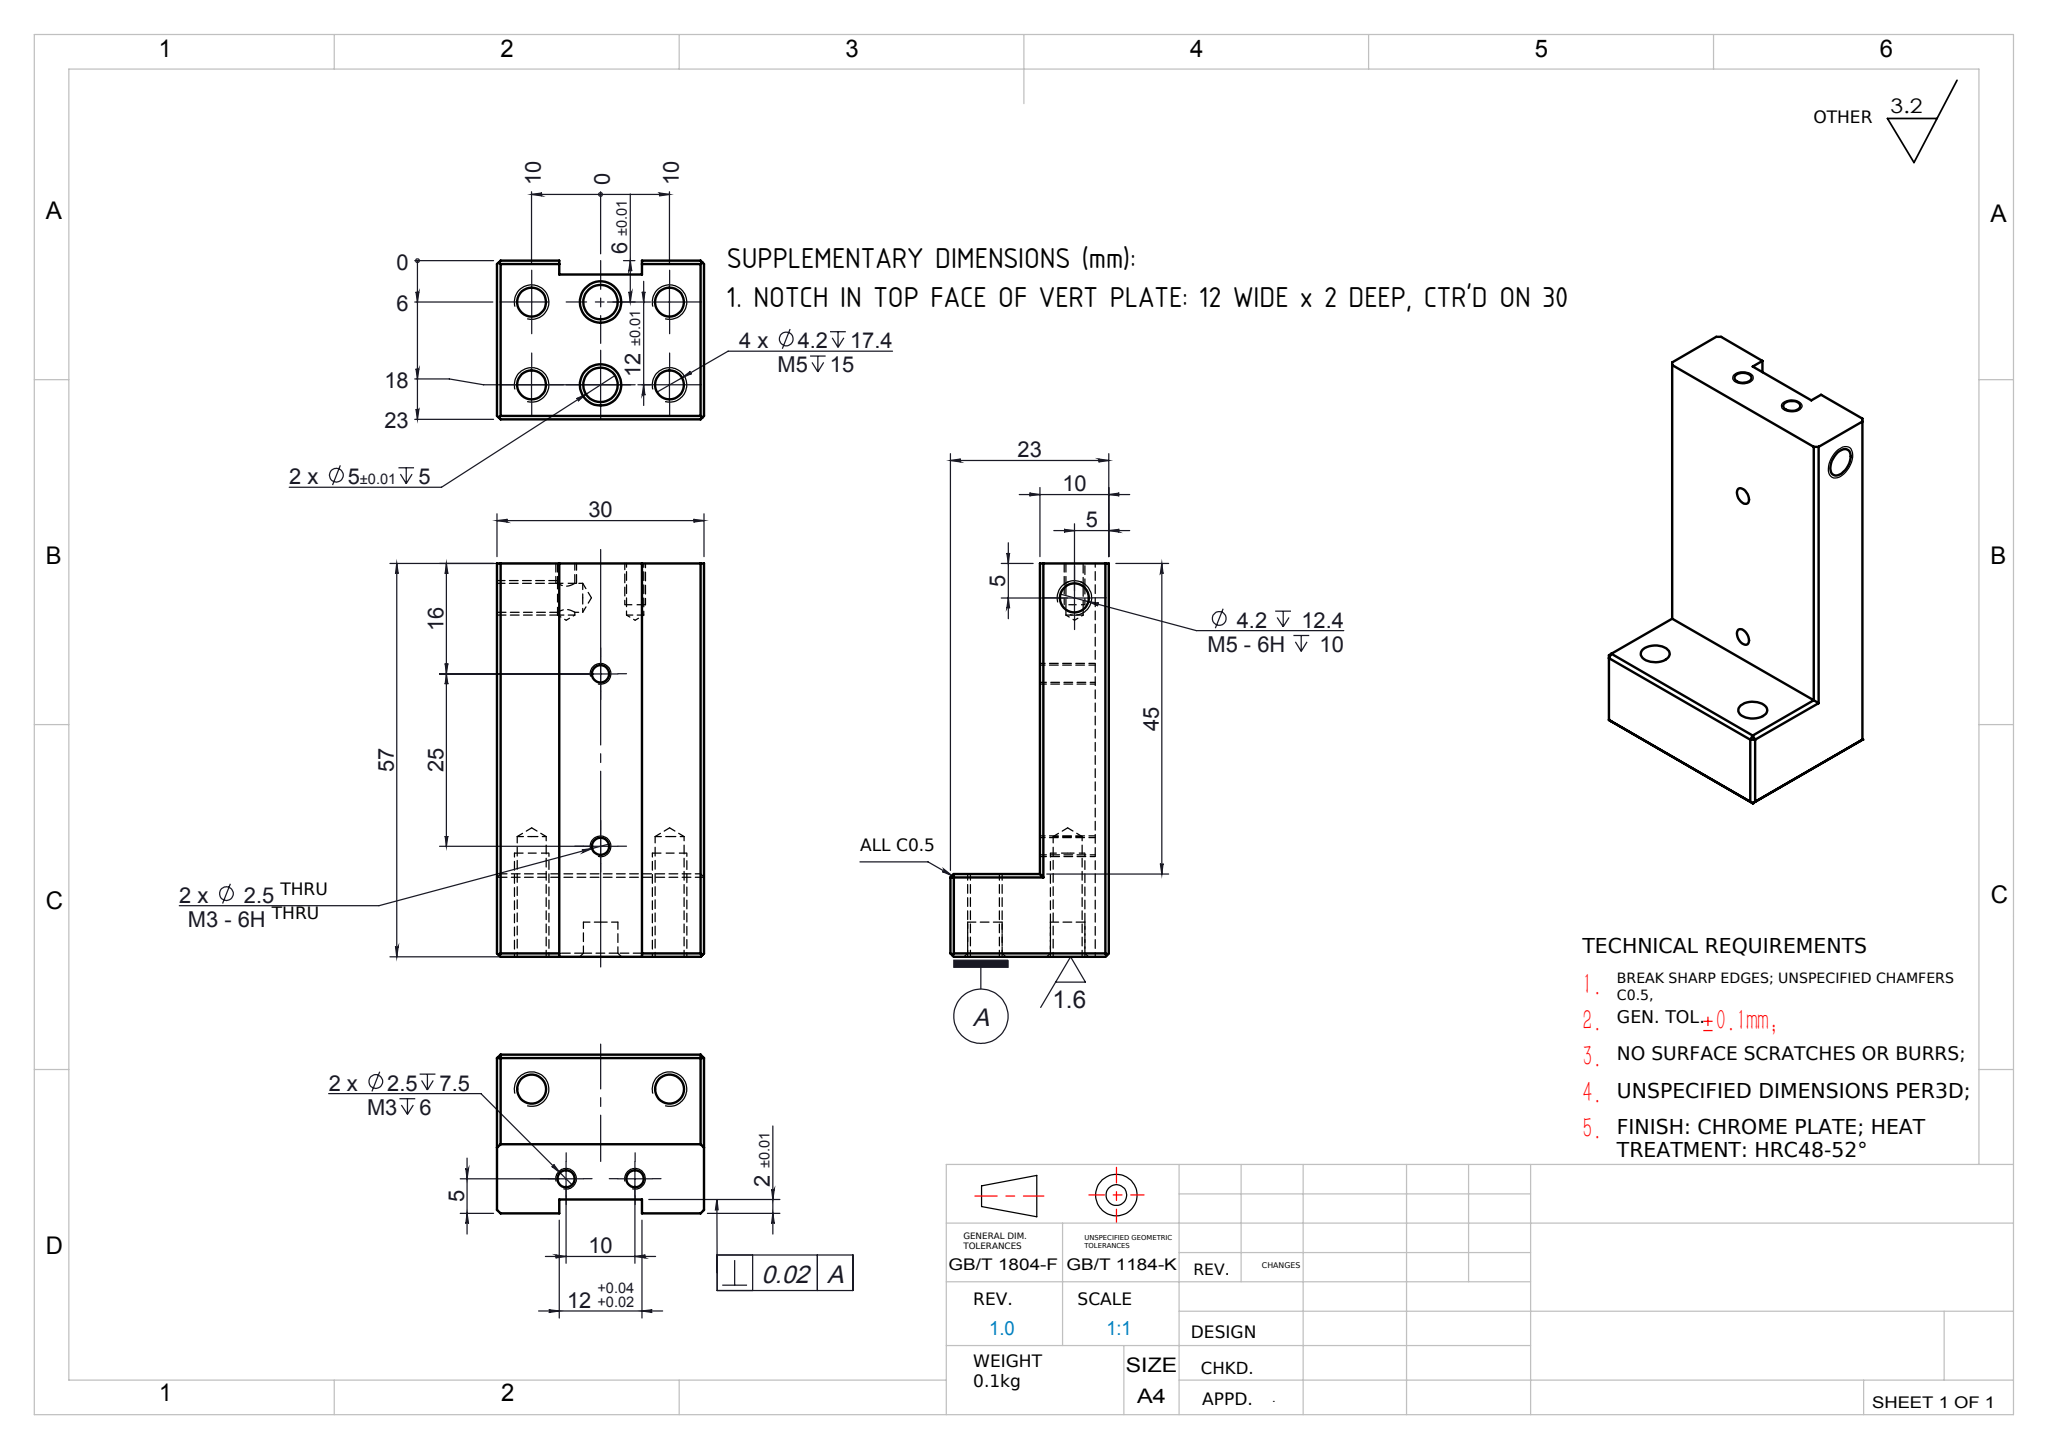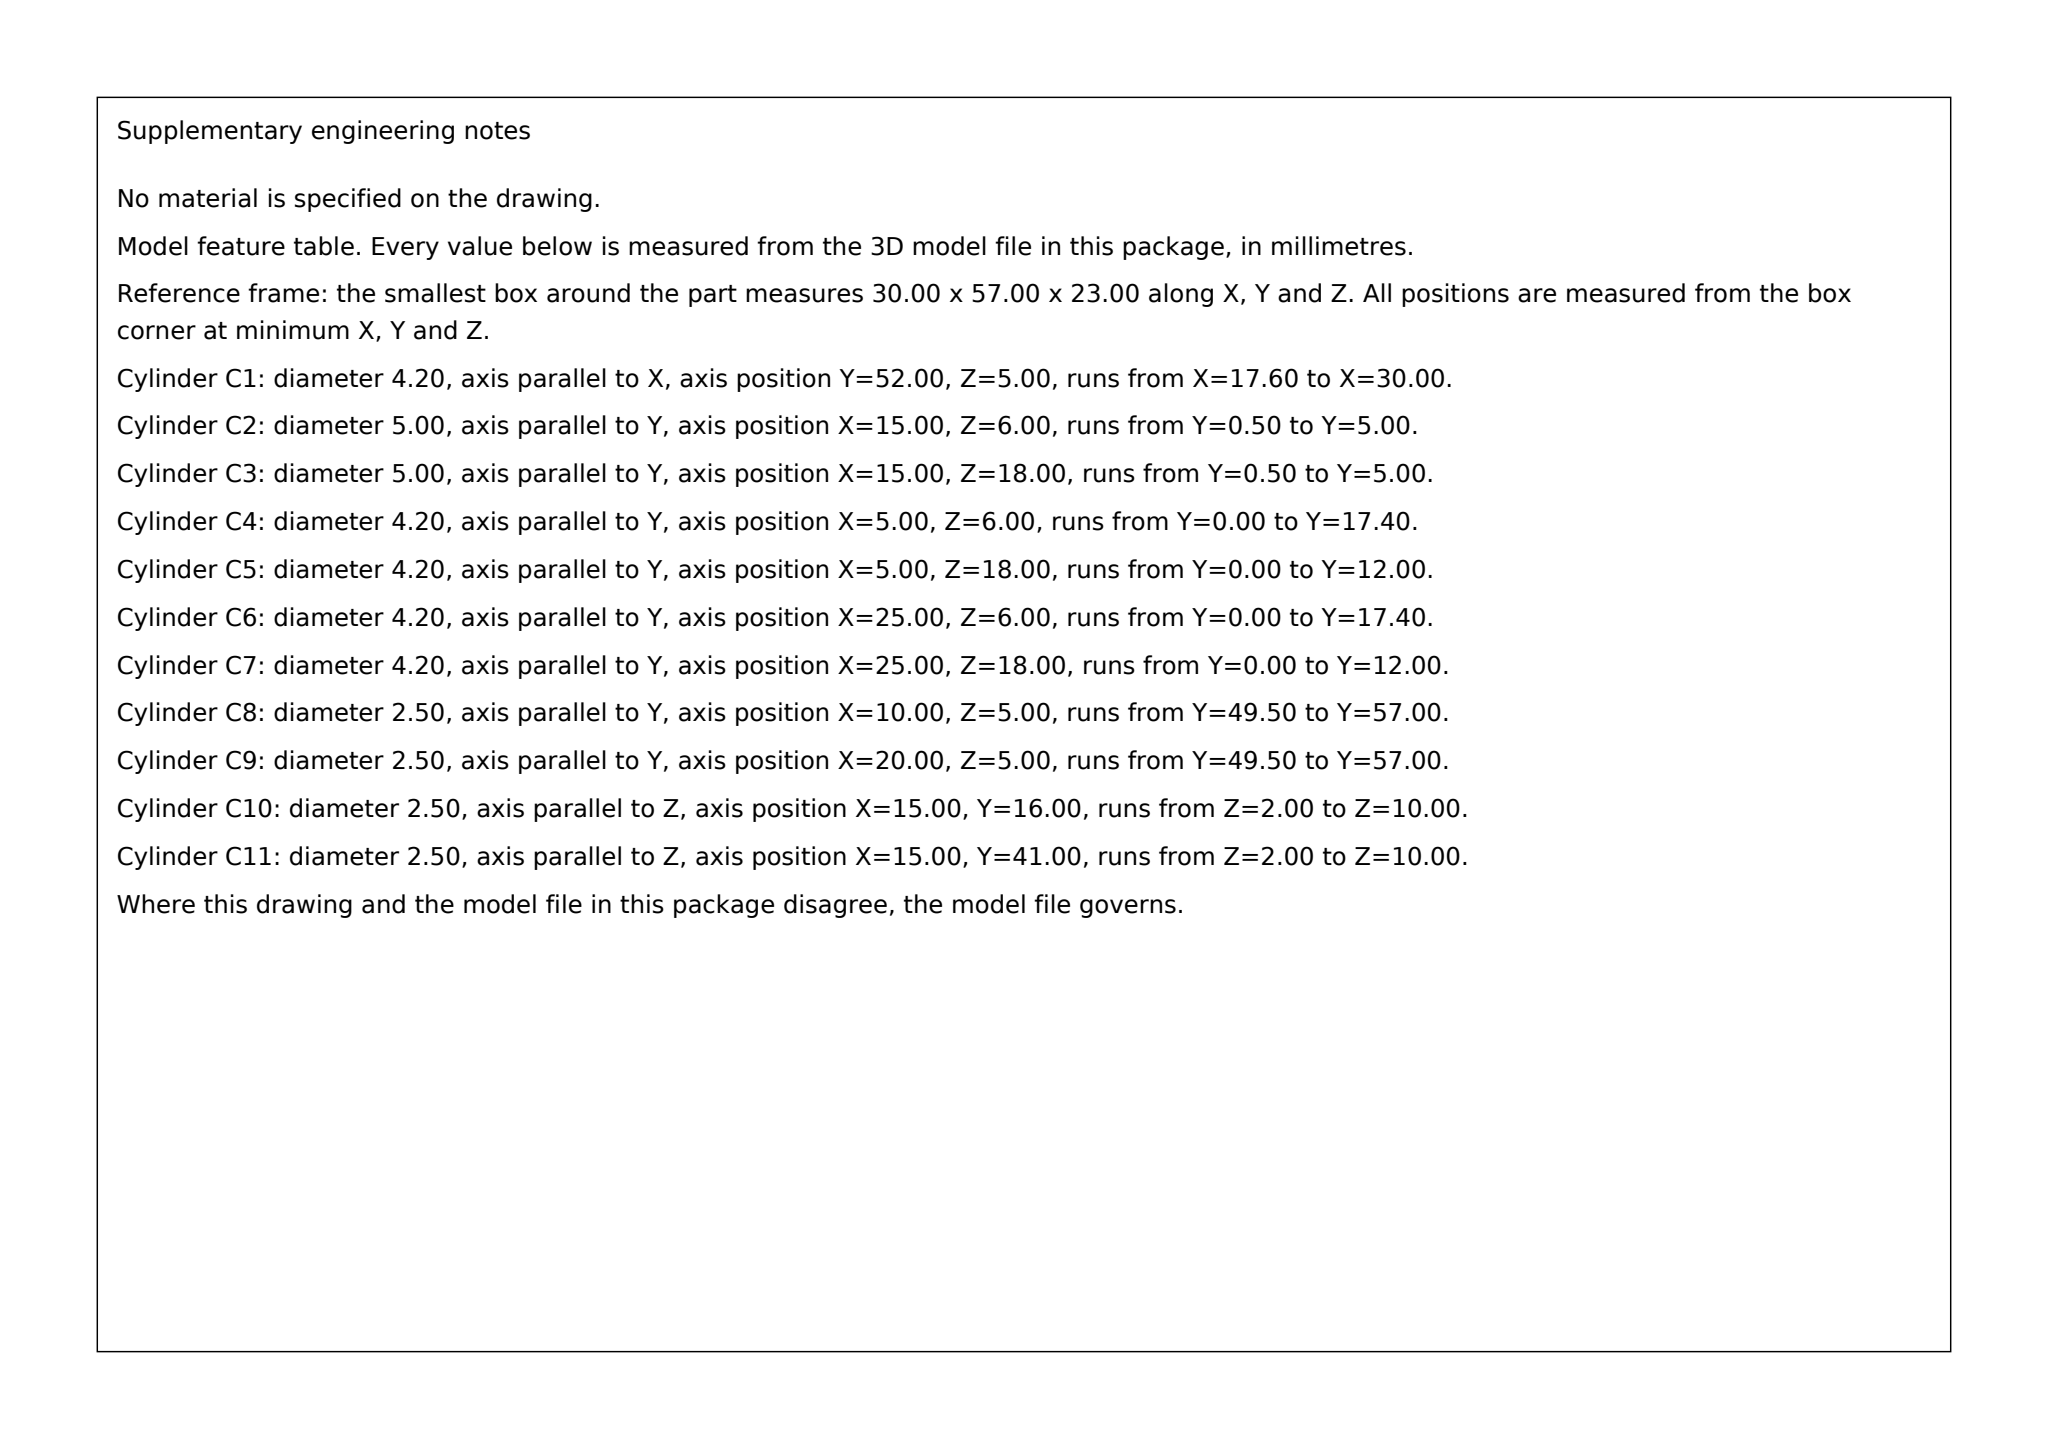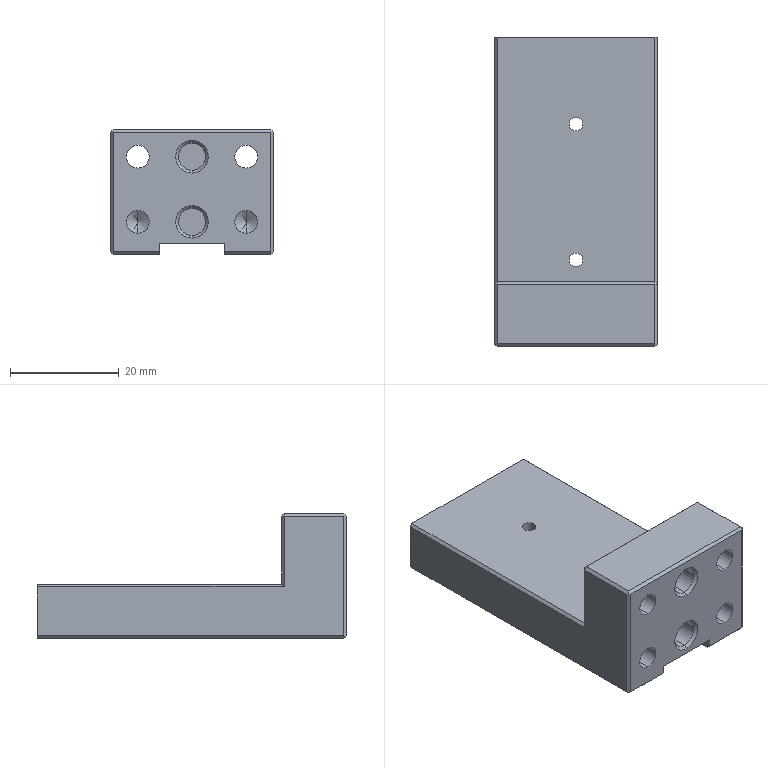Part | SolidWorks | mm | 1 solid | 68 faces | box 30 x 57 x 23 mm | volume 19026 mm3 | plane 30 | cylinder 24 | cone 14 | commonest cylinder face diameters 4.2 x10 2.5 x10 5 x4